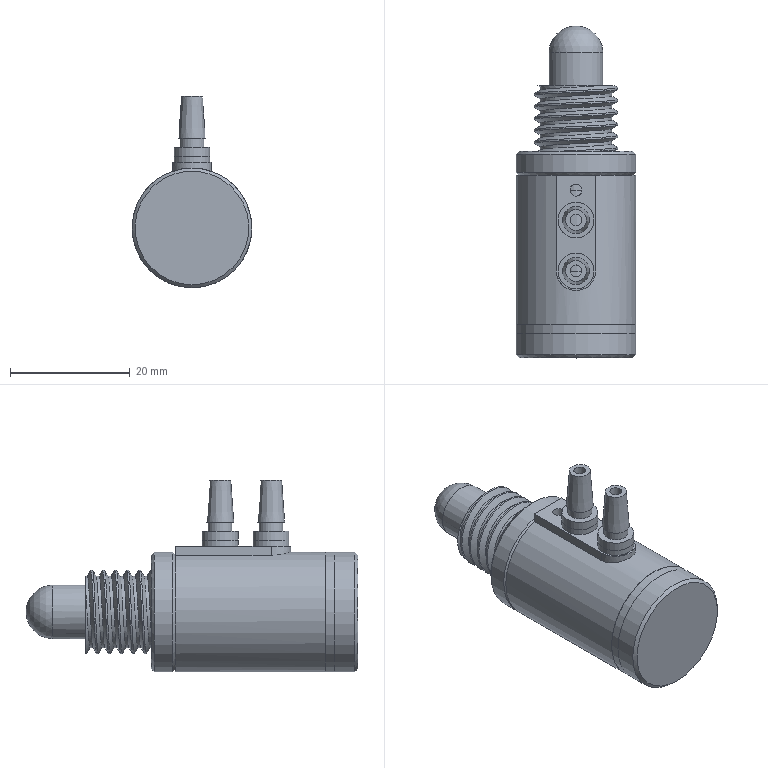Assembly | NX | mm | 11 component files | 11 solids | 108 faces | box 20 x 55.45 x 32 mm | volume 11469 mm3 | cylinder 49 | plane 43 | spline 8 | cone 5 | torus 2 | sphere 1 | commonest cylinder face diameters 14 x11 4 x9 6 x5 20 x4 2 x3 5 x3 9 x2 3.5 x2
Bill of materials:
unnamed part 1 | 1 |  | Stepped cylindrical body with a bore that has internal threads at one end and a smaller-diameter, externally threaded spigot at the other. A raised flat pad with rounded ends runs along the outer surface and has two threaded holes plus one small plain hole.
unnamed part 2 | 2 |  | Flat annular ring (washer-like) with a rectangular cross-section, plain cylindrical inner and outer faces, and flat parallel faces.
unnamed part 3 | 2 |  | Hollow, axially symmetric stepped tube. It has a tapered conical section at one end, a short cylindrical neck, a thin radial collar, a reduced groove-like step, and a plain cylindrical section at the other end.
unnamed part 4 | 1 |  | Thin flat annular ring with a wide hole relative to its outer diameter and a small, constant thickness.
unnamed part 5 | 1 |  | Slender torus (round-section ring) with a small cross-section compared with its overall diameter.
unnamed part 6 | 1 |  | Thick annular ring with a rectangular cross-section and small chamfers on the outer edges of both faces.
unnamed part 7 | 1 |  | Solid stepped cylindrical plug or cap shape. It has a large-diameter disk-shaped head with a chamfered edge, a short reduced-diameter neck forming a groove, and a cylindrical boss of intermediate diameter.
unnamed part 8 | 1 |  | Long, slender, stepped cylindrical pin. One end is a long main shank with a rounded, domed tip. Moving toward the other end it has a narrow groove, a shorter cylindrical section of slightly smaller diameter, a thin radial flange, and a small-diameter stub projecting beyond the flange.
unnamed part 9 | 1 |  | Torus (round-section ring) with a thick cross-section compared with its overall diameter, leaving a fairly small central hole.
Mates:
1. touch align | end_cap 1 face | valve_body 1 face
2. touch align | large_washer 1 face | end_cap 1 face
3. touch align | pipe_joint 2 face | valve_body 1 face
4. touch align | small_washer 2 face | pipe_joint 2 face
5. touch align | small_washer 2 face | pipe_joint 2 face
6. touch align | small_washer 2 face | valve_body 1 face
7. touch align | nut 1 face | end_cap 1 face
8. touch align | valve_core 1 face | nut 1 face
9. touch align | o_ring 1 face | valve_core 1 face
10. touch align | o_ring_2 1 face | o_ring 1 face
11. touch align | nut 1 face | valve_body 1 face
12. touch align | valve_body 1 face | large_washer 1 face
13. touch align | large_washer 1 face | end_cap 1 face
14. touch align | small_washer 1 face | pipe_joint 1 face
15. touch align | pipe_joint 1 face | small_washer 1 face